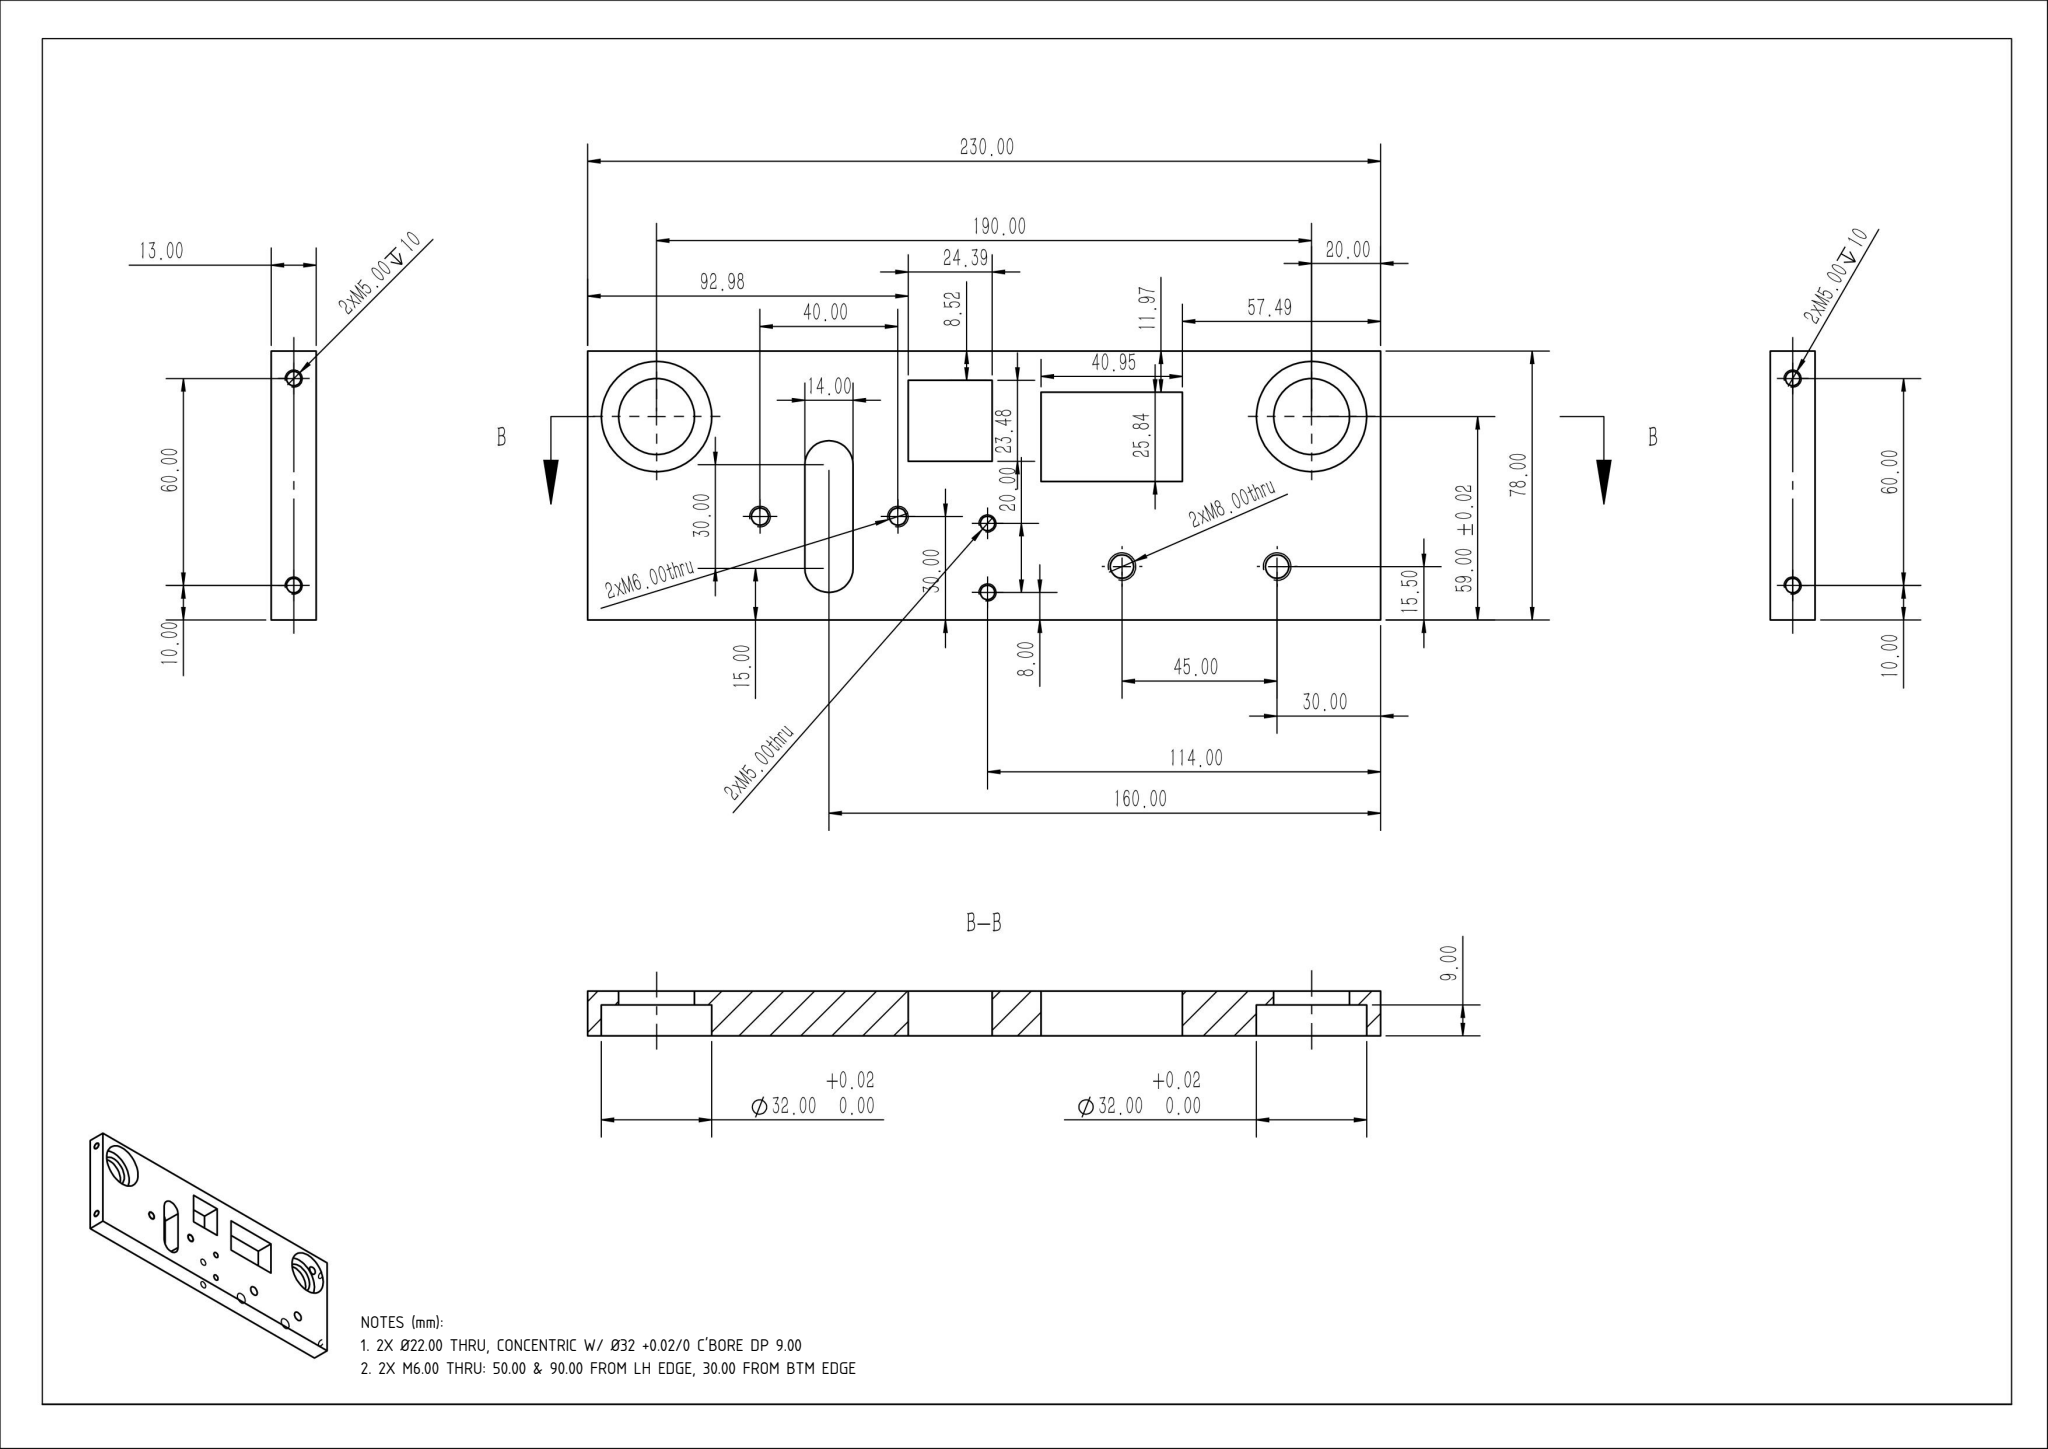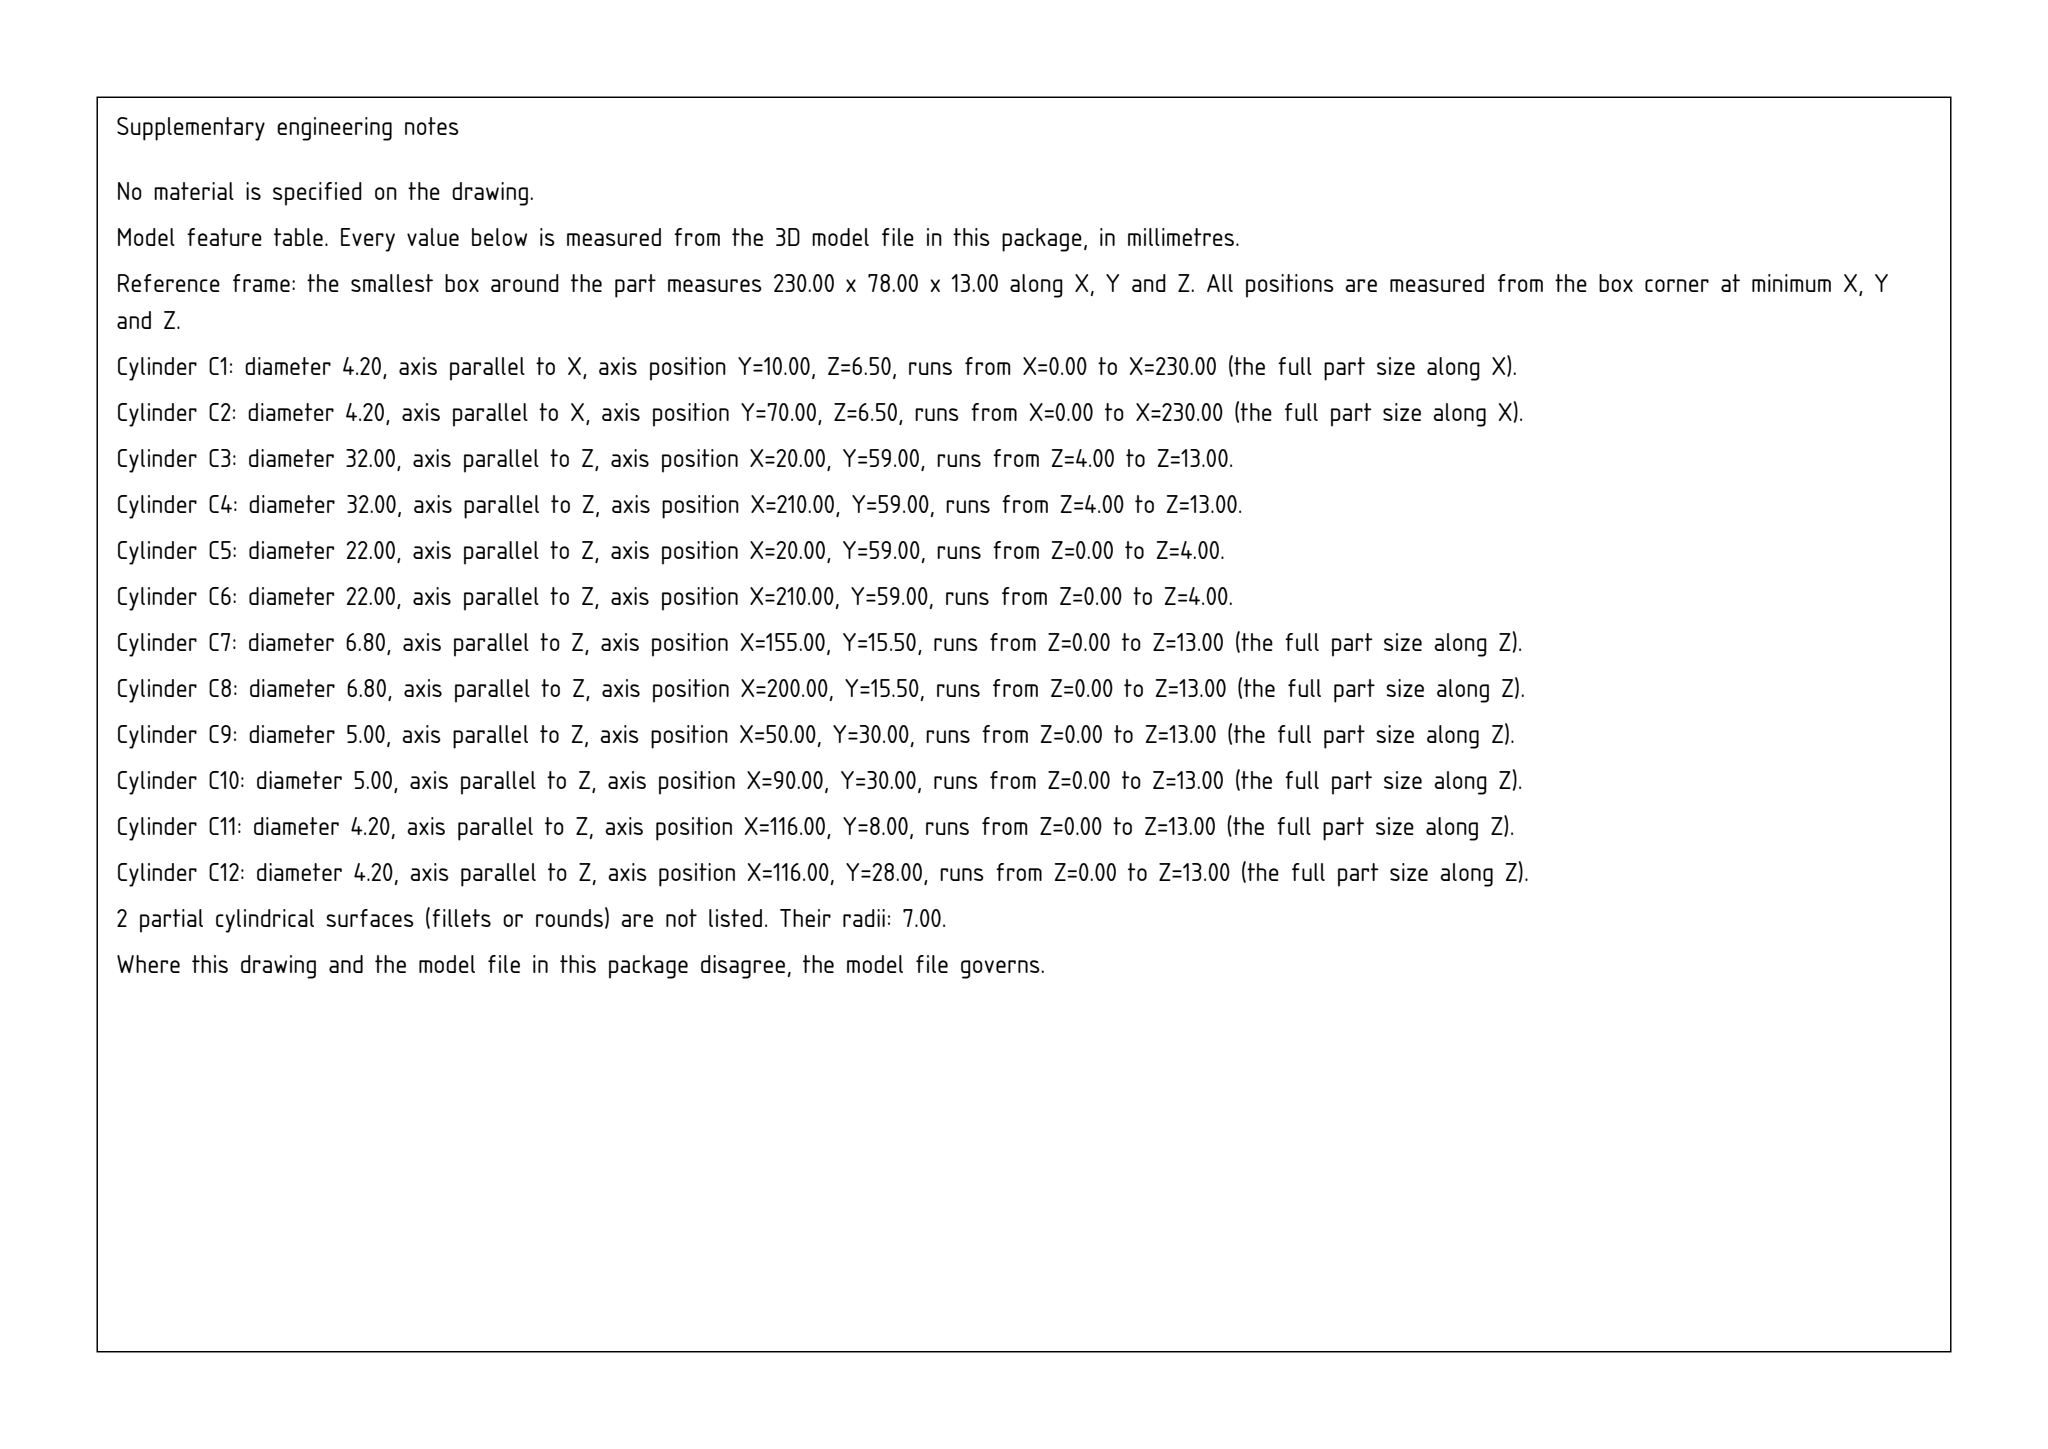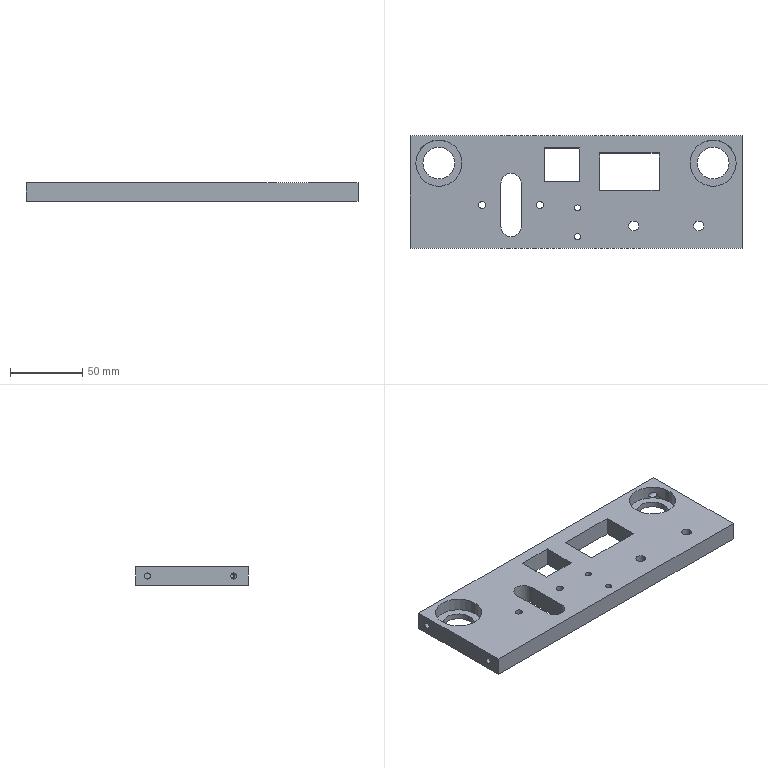Part | SolidWorks | mm | 1 solid | 52 faces | box 230 x 78 x 13 mm | volume 184636 mm3 | cylinder 30 | plane 18 | cone 4 | commonest cylinder face diameters 4.2 x12 6.8 x4 5 x4 32 x4 22 x4 14 x2
Drawing notes:
2X Ø22.00 THRU, CONCENTRIC W/ Ø32 +0.02/0 C'BORE DP 9.00 | from the solid: cylinders dia 22.0 axis z at [20,59] and [210,59], len 4.0 under dia 32.0 len 9.0 same axes; plate thk 13.0
2X M6.00 THRU: 50.00 & 90.00 FROM LH EDGE, 30.00 FROM BTM EDGE | from the solid: cylinders dia 5.0 z-axis at (50,30) and (90,30), bbox 230x78x13 from min corner
build123d program:
from build123d import *

# Parameters (mm, degrees)
SKETCH1_W             = 230
SKETCH1_H             = 78
BOSS_EXTRUDE1_DEPTH   = 6.5
SKETCH2_R             = 11
CUT_EXTRUDE1_DEPTH    = 244.214
SKETCH3_R             = 16
CUT_EXTRUDE2_DEPTH    = 9
CUT_EXTRUDE3_DEPTH    = 244.214
M6_TAPPED_HOLE1_D     = 5
M8_TAPPED_HOLE1_D     = 6.8
M5_TAPPED_HOLE1_D     = 4.2
M5_TAPPED_HOLE1_DEPTH = 12.4
M5_TAPPED_HOLE1_TIP   = 1.262
M5_TAPPED_HOLE2_D     = 4.2
M5_TAPPED_HOLE2_DEPTH = 12.4
M5_TAPPED_HOLE2_TIP   = 1.262
M5_TAPPED_HOLE3_D     = 4.2
SKETCH18_W            = 24.387
SKETCH18_H            = 23.477
SKETCH18_W_2          = 40.948
SKETCH18_H_2          = 25.843
CUT_EXTRUDE4_DEPTH    = 78


with BuildPart() as part:
    # Sketch1 → Boss-Extrude1 (new, symmetric)
    with BuildSketch(Plane.XY):
        with Locations((-115, 39)):
            Rectangle(SKETCH1_W, SKETCH1_H)
    extrude(amount=BOSS_EXTRUDE1_DEPTH, both=True)

    # Sketch2 → Cut-Extrude1 (cut, through all)
    with BuildSketch(Plane.XY.offset(6.5)):
        with Locations((-20, 59)):
            Circle(SKETCH2_R)
        with Locations((-210, 59)):
            Circle(SKETCH2_R)
    extrude(amount=-CUT_EXTRUDE1_DEPTH, mode=Mode.SUBTRACT)

    # Sketch3 → Cut-Extrude2 (cut)
    with BuildSketch(Plane.XY.offset(6.5)):
        with Locations((-20, 59)):
            Circle(SKETCH3_R)
        with Locations((-210, 59)):
            Circle(SKETCH3_R)
    extrude(amount=-CUT_EXTRUDE2_DEPTH, mode=Mode.SUBTRACT)

    # Sketch5 → Cut-Extrude3 (cut, through all)
    with BuildSketch(Plane.XY.offset(6.5)):
        with BuildLine():
            Line((-153, 45), (-153, 15))
            ThreePointArc((-153, 15), (-160, 8), (-167, 15))
            Line((-167, 15), (-167, 45))
            ThreePointArc((-167, 45), (-160, 52), (-153, 45))
        make_face()
    extrude(amount=-CUT_EXTRUDE3_DEPTH, mode=Mode.SUBTRACT)

    # M6 Tapped Hole1 (through all)
    with Locations(Plane.XY.offset(6.5)):
        with Locations((-180, 30), (-140, 30)):
            Hole(M6_TAPPED_HOLE1_D / 2)

    # M8 Tapped Hole1 (through all)
    with Locations(Plane(origin=(0, 0, -6.5), x_dir=(-1, 0, 0), z_dir=(0, 0, -1))):
        with Locations((30, 15.5), (75, 15.5)):
            Hole(M8_TAPPED_HOLE1_D / 2)

    # M5 Tapped Hole1
    with Locations(Plane.ZY.offset(230)):
        with Locations((0, 70), (0, 10)):
            Hole(M5_TAPPED_HOLE1_D / 2, depth=M5_TAPPED_HOLE1_DEPTH)
            with Locations((0, 0, -(M5_TAPPED_HOLE1_DEPTH + M5_TAPPED_HOLE1_TIP / 2))):  # 118° drill point
                Cone(0, M5_TAPPED_HOLE1_D / 2, M5_TAPPED_HOLE1_TIP, mode=Mode.SUBTRACT)

    # M5 Tapped Hole2
    with Locations(Plane(origin=(0, 0, 0), x_dir=(0, 0, -1), z_dir=(1, 0, 0))):
        with Locations((0, 70), (0, 10)):
            Hole(M5_TAPPED_HOLE2_D / 2, depth=M5_TAPPED_HOLE2_DEPTH)
            with Locations((0, 0, -(M5_TAPPED_HOLE2_DEPTH + M5_TAPPED_HOLE2_TIP / 2))):  # 118° drill point
                Cone(0, M5_TAPPED_HOLE2_D / 2, M5_TAPPED_HOLE2_TIP, mode=Mode.SUBTRACT)

    # M5 Tapped Hole3 (through all)
    with Locations(Plane(origin=(0, 0, -6.5), x_dir=(-1, 0, 0), z_dir=(0, 0, -1))):
        with Locations((114, 28), (114, 8)):
            Hole(M5_TAPPED_HOLE3_D / 2)

    # Sketch18 → Cut-Extrude4 (cut)
    with BuildSketch(Plane.XY.offset(6.5)):
        with Locations((-124.828, 57.745)):
            Rectangle(SKETCH18_W, SKETCH18_H)
        with Locations((-77.964, 53.104)):
            Rectangle(SKETCH18_W_2, SKETCH18_H_2)
    extrude(amount=-CUT_EXTRUDE4_DEPTH, mode=Mode.SUBTRACT)


solid = part.part